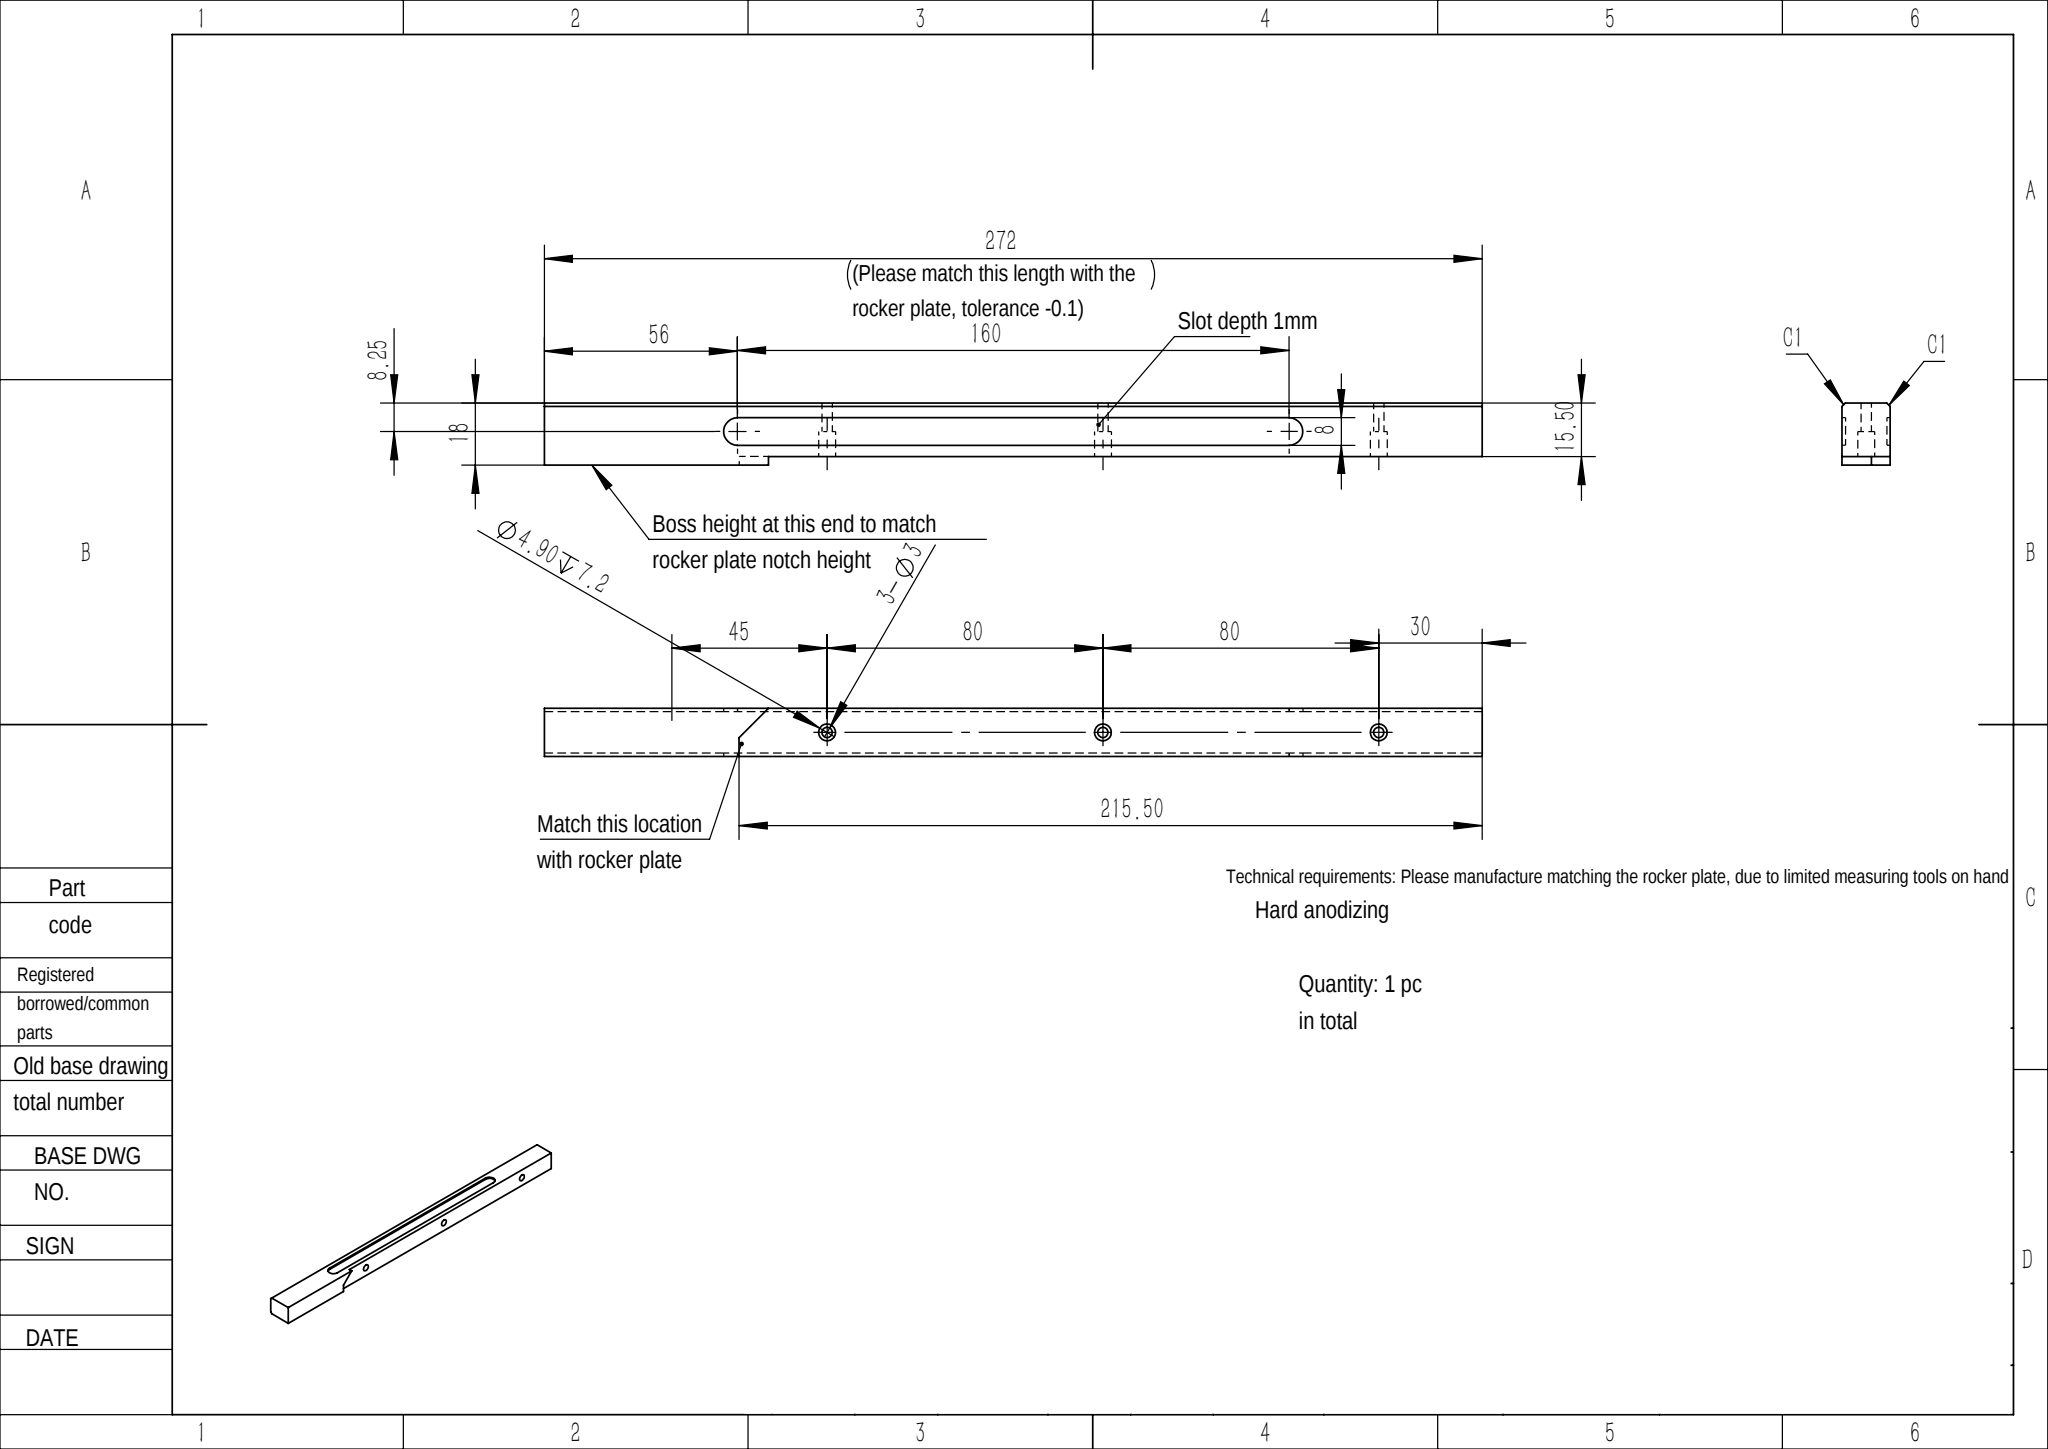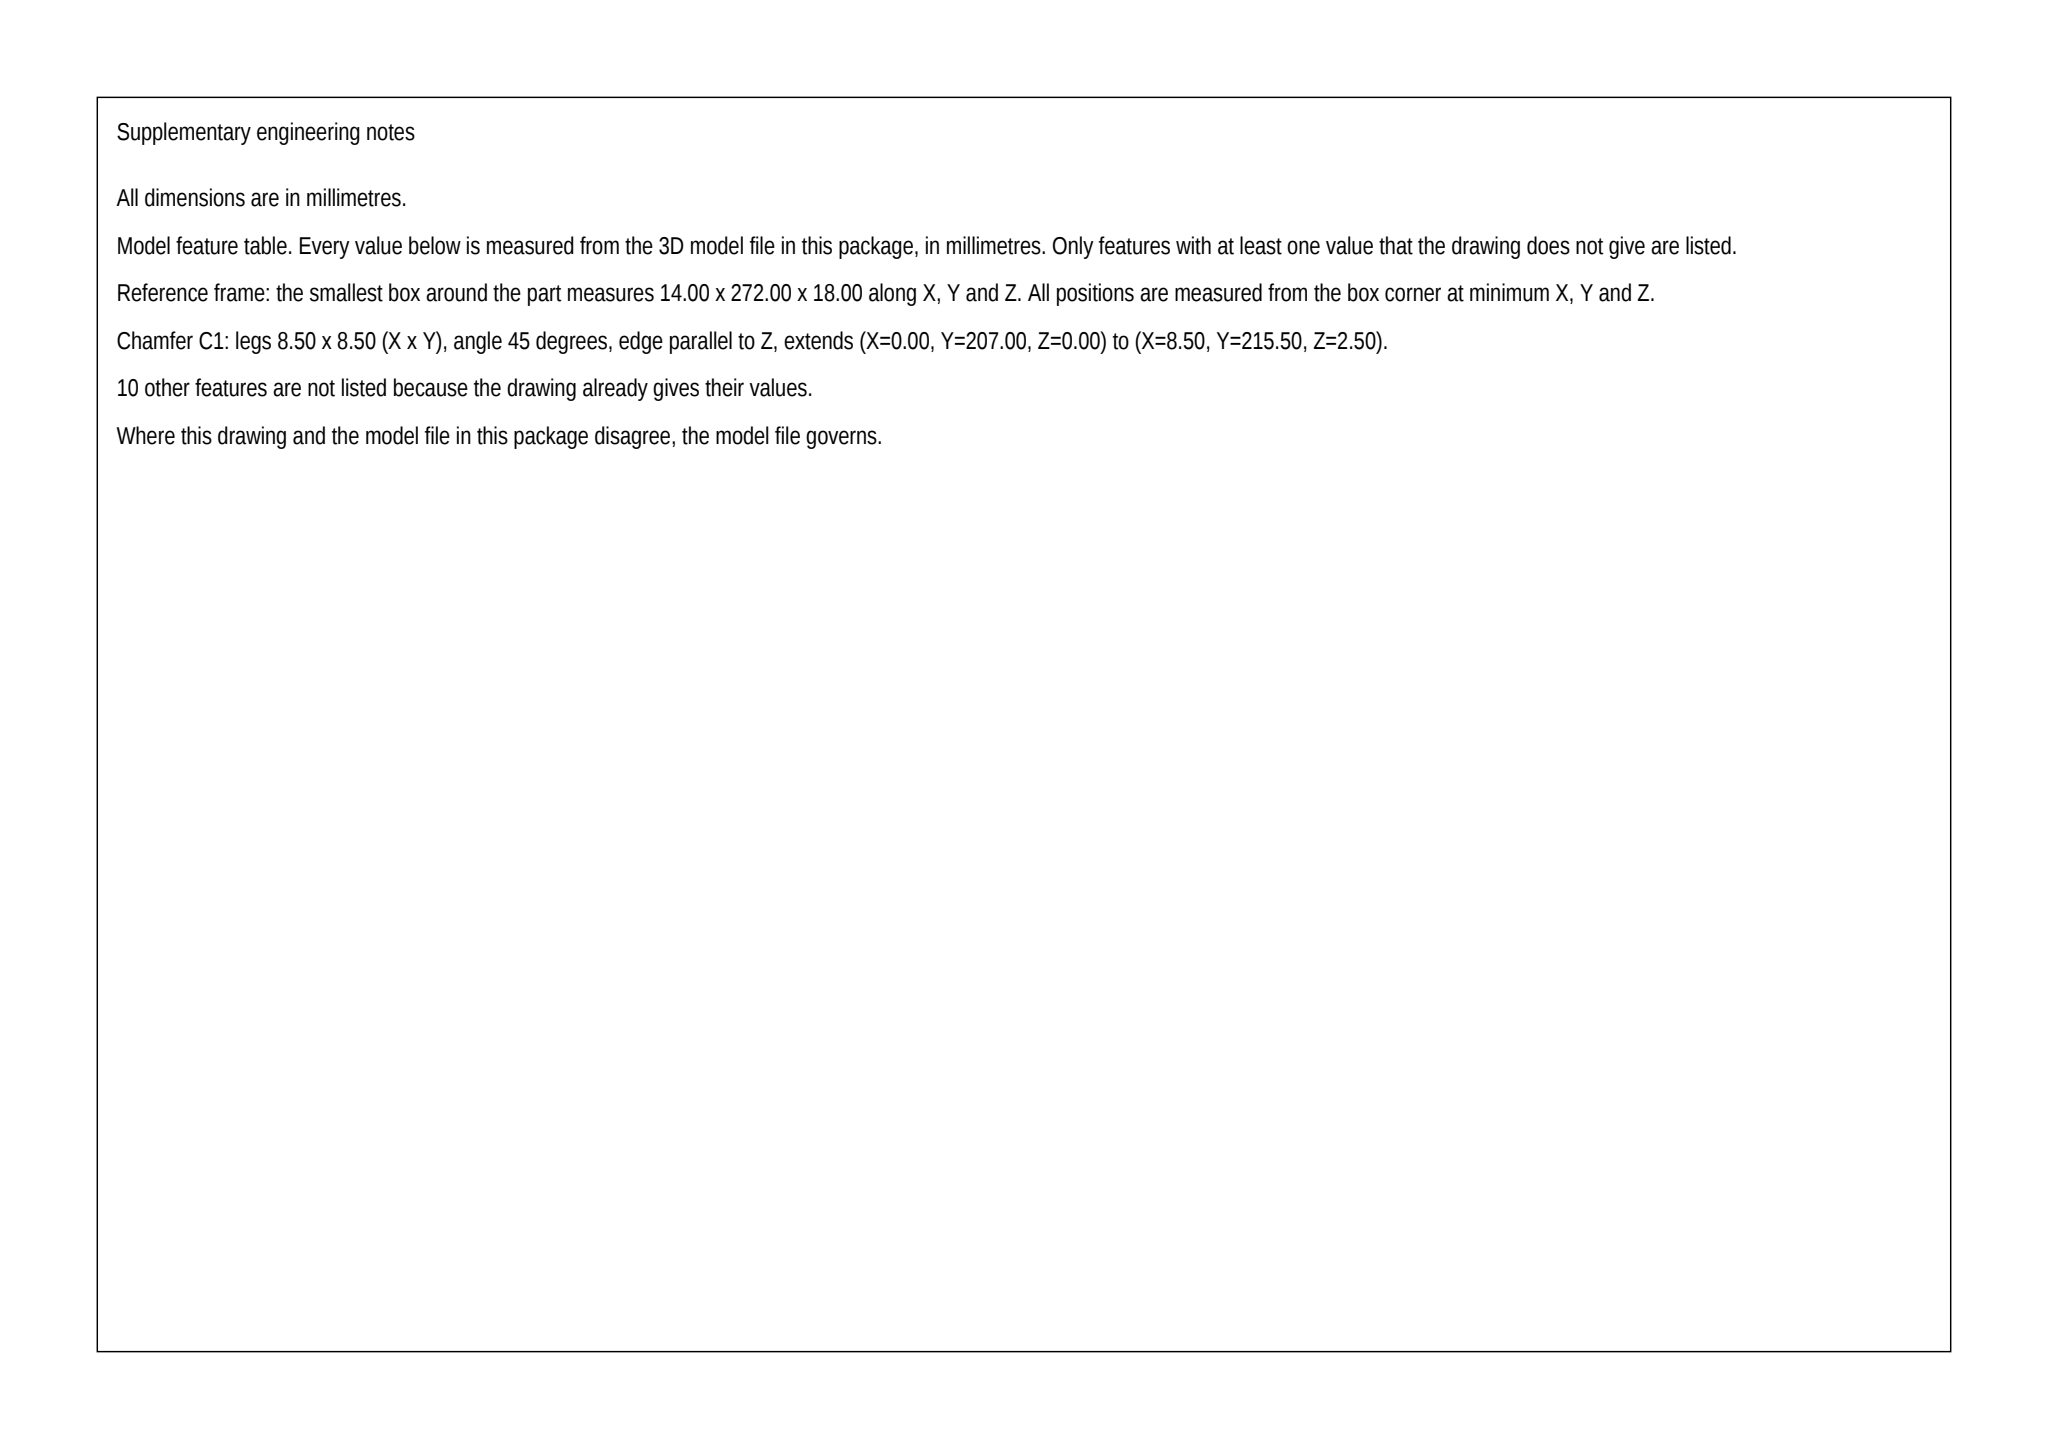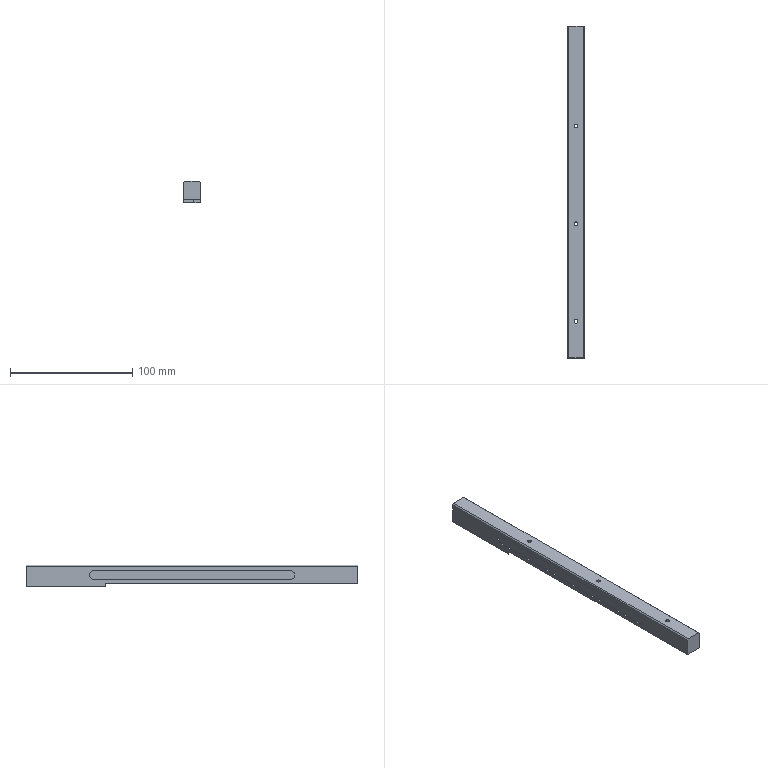Part | SolidWorks | mm | 1 solid | 38 faces | box 14 x 272 x 18 mm | volume 57576 mm3 | plane 20 | cylinder 18 | commonest cylinder face diameters 8 x6 3 x6 4.9 x6
Drawing notes:
BOSS AT LH END: 12 WIDE, 1 RELIEF EA SIDE (BAR 14 WIDE) | from the solid: x planes at 0,1,13,14; reduced section between x=1 and x=13 = 12 wide, bbox x=14
BOSS 2.5 HIGH x 56.5 LG FROM LH END TO STEP FACE | from the solid: z planes 0 & 2.5; y planes 215.5 & 272 -> 272-215.5=56.5 step length, step face at 215.50 from RH end
HOLE CHAIN DATUM RH END: Ø3 C/L AT 30, 110 & 190 | from the solid: Ø3/Ø4.9 cyl axes at y=30, 110, 190 from y=0 (RH end); closes with 272 overall
build123d program:
from build123d import *

# Parameters (mm, degrees)
SKETCH1_W           = 14
SKETCH1_H           = 272
BOSS_EXTRUDE1_DEPTH = 15.5
SKETCH2_W           = 14
SKETCH2_H           = 56.5
BOSS_EXTRUDE2_DEPTH = 2.5
SKETCH3_R           = 2.45
CUT_EXTRUDE1_DEPTH  = 7.2
LPATTERN1_COUNT     = 3
LPATTERN1_PITCH     = 80
SKETCH4_R           = 1.5
CUT_EXTRUDE2_DEPTH  = 138.059
LPATTERN2_COUNT     = 3
LPATTERN2_PITCH     = 80
CHAMFER1_SIZE       = 1
CUT_EXTRUDE3_DEPTH  = 1
BOSS_EXTRUDE3_DEPTH = 2.5


with BuildPart() as part:
    # Sketch1 → Boss-Extrude1 (new body)
    with BuildSketch(Plane.XY):
        Rectangle(SKETCH1_W, SKETCH1_H)
    extrude(amount=BOSS_EXTRUDE1_DEPTH)

    # Sketch2 → Boss-Extrude2 (add)
    with BuildSketch(Plane(origin=(0, 0, 0), x_dir=(-1, 0, 0), z_dir=(0, 0, -1))):
        with Locations((0, 107.75)):
            Rectangle(SKETCH2_W, SKETCH2_H)
    extrude(amount=BOSS_EXTRUDE2_DEPTH)

    # Sketch3 → Cut-Extrude1 (cut)
    with BuildSketch(Plane(origin=(0, 0, 0), x_dir=(-1, 0, 0), z_dir=(0, 0, -1))):
        with Locations((0, -106)):
            Circle(SKETCH3_R)
    cut_extrude1 = extrude(amount=-CUT_EXTRUDE1_DEPTH, mode=Mode.SUBTRACT)

    # LPattern1: Cut-Extrude1 ×3
    with Locations(*[(0, i * LPATTERN1_PITCH, 0) for i in range(1, LPATTERN1_COUNT)]):
        add(cut_extrude1, mode=Mode.SUBTRACT)

    # Sketch4 → Cut-Extrude2 (cut, through all)
    with BuildSketch(Plane(origin=(0, 0, 0), x_dir=(-1, 0, 0), z_dir=(0, 0, -1))):
        with Locations((0, -106)):
            Circle(SKETCH4_R)
    cut_extrude2 = extrude(amount=-CUT_EXTRUDE2_DEPTH, mode=Mode.SUBTRACT)

    # LPattern2: Cut-Extrude2 ×3
    with Locations(*[(0, i * LPATTERN2_PITCH, 0) for i in range(1, LPATTERN2_COUNT)]):
        add(cut_extrude2, mode=Mode.SUBTRACT)

    # Chamfer1
    chamfer1_edges = [part.edges().sort_by_distance(p)[0] for p in [
        (-7, 0, 15.5),
        (7, 0, 15.5),
    ]]
    chamfer(chamfer1_edges, length=CHAMFER1_SIZE)

    # Sketch5 → Cut-Extrude3 (cut)
    with BuildSketch(Plane(origin=(7, 0, 0), x_dir=(0, 0, -1), z_dir=(1, 0, 0))):
        with BuildLine():
            Line((-11.25, -80), (-11.25, 80))
            ThreePointArc((-11.25, 80), (-7.25, 84), (-3.25, 80))
            Line((-3.25, 80), (-3.25, -80))
            ThreePointArc((-3.25, -80), (-7.25, -84), (-11.25, -80))
        make_face()
    cut_extrude3 = extrude(amount=-CUT_EXTRUDE3_DEPTH, mode=Mode.SUBTRACT)

    # Mirror1: Cut-Extrude3 across plane
    add(cut_extrude3.mirror(Plane(origin=(0, 0, 0), x_dir=(0, 0, 1), z_dir=(1, 0, 0))), mode=Mode.SUBTRACT)

    # Sketch6 → Boss-Extrude3 (add)
    with BuildSketch(Plane(origin=(0, 0, 0), x_dir=(-1, 0, 0), z_dir=(0, 0, -1))):
        Polygon((-1.5, 79.5), (7, 71), (7, 79.5), align=None)
    extrude(amount=BOSS_EXTRUDE3_DEPTH)


solid = part.part